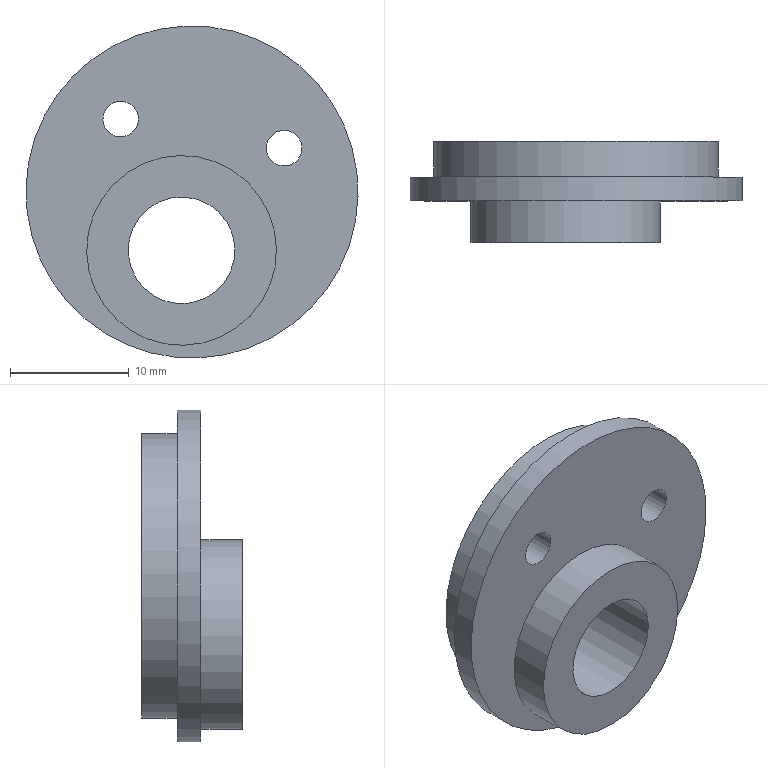Component | NX | ECCENTRIC | 1 solid | 10 faces | box 28 x 8.5 x 28 mm | volume 2681 mm3 | cylinder 6 | plane 4 | commonest cylinder face diameters 3 x2 24 x1 28 x1 16 x1 9 x1
STEP:
#1=CARTESIAN_POINT('',(0.,0.,0.));
#2=DIRECTION('',(0.,0.,1.));
#3=DIRECTION('',(1.,0.,0.));
#4=AXIS2_PLACEMENT_3D('',#1,#2,#3);
#5=CARTESIAN_POINT('',(56.622,60.5,26.855));
#6=VERTEX_POINT('',#5);
#7=CARTESIAN_POINT('',(53.668,60.5,27.381));
#8=VERTEX_POINT('',#7);
#9=CARTESIAN_POINT('',(55.145,60.5,27.118));
#10=DIRECTION('',(0.,-1.,0.));
#11=DIRECTION('',(0.9845,0.,-0.1753));
#12=AXIS2_PLACEMENT_3D('',#9,#10,#11);
#13=CIRCLE('',#12,1.5);
#14=CARTESIAN_POINT('',(47.377,60.5,23.423));
#15=DIRECTION('',(0.,1.,0.));
#16=DIRECTION('',(0.9845,0.,-0.1753));
#17=AXIS2_PLACEMENT_3D('',#14,#15,#16);
#18=PLANE('',#17);
#19=CARTESIAN_POINT('',(8.5,-5.));
#20=CARTESIAN_POINT('',(8.5,-7.598));
#21=CARTESIAN_POINT('',(6.25,-6.299));
#22=CARTESIAN_POINT('',(4.,-5.));
#23=CARTESIAN_POINT('',(6.25,-3.701));
#24=CARTESIAN_POINT('',(8.5,-2.402));
#25=CARTESIAN_POINT('',(8.5,-5.));
#26=(BOUNDED_CURVE()B_SPLINE_CURVE(2,(#19,#20,#21,#22,#23,#24,#25),.UNSPECIFIED.,.T.,.F.)B_SPLINE_CURVE_WITH_KNOTS((1,2,2,2,2,1),(-2.094,0.,2.094,4.189,6.283,8.378),.UNSPECIFIED.)CURVE()GEOMETRIC_REPRESENTATION_ITEM()RATIONAL_B_SPLINE_CURVE((1.,0.5,1.,0.5,1.,0.5,1.))REPRESENTATION_ITEM(''));
#27=(GEOMETRIC_REPRESENTATION_CONTEXT(2)PARAMETRIC_REPRESENTATION_CONTEXT()REPRESENTATION_CONTEXT('',''));
#28=DEFINITIONAL_REPRESENTATION('',(#26),#27);
#29=PCURVE('',#18,#28);
#30=CARTESIAN_POINT('',(55.145,72.,27.118));
#31=DIRECTION('',(0.,-1.,0.));
#32=DIRECTION('',(-0.9845,0.,0.1753));
#33=AXIS2_PLACEMENT_3D('',#30,#31,#32);
#34=CYLINDRICAL_SURFACE('',#33,1.5);
#35=CARTESIAN_POINT('',(3.142,11.5));
#36=DIRECTION('',(1.,0.));
#37=VECTOR('',#36,1.);
#38=LINE('',#35,#37);
#39=(GEOMETRIC_REPRESENTATION_CONTEXT(2)PARAMETRIC_REPRESENTATION_CONTEXT()REPRESENTATION_CONTEXT('',''));
#40=DEFINITIONAL_REPRESENTATION('',(#38),#39);
#41=PCURVE('',#34,#40);
#42=SURFACE_CURVE('',#13,(#29,#41),.PCURVE_S1.);
#43=EDGE_CURVE('',#6,#8,#42,.T.);
#44=ORIENTED_EDGE('',*,*,#43,.T.);
#45=CARTESIAN_POINT('',(55.145,60.5,27.118));
#46=DIRECTION('',(0.,-1.,0.));
#47=DIRECTION('',(0.9845,0.,-0.1753));
#48=AXIS2_PLACEMENT_3D('',#45,#46,#47);
#49=CIRCLE('',#48,1.5);
#50=CARTESIAN_POINT('',(8.5,-5.));
#51=CARTESIAN_POINT('',(8.5,-7.598));
#52=CARTESIAN_POINT('',(6.25,-6.299));
#53=CARTESIAN_POINT('',(4.,-5.));
#54=CARTESIAN_POINT('',(6.25,-3.701));
#55=CARTESIAN_POINT('',(8.5,-2.402));
#56=CARTESIAN_POINT('',(8.5,-5.));
#57=(BOUNDED_CURVE()B_SPLINE_CURVE(2,(#50,#51,#52,#53,#54,#55,#56),.UNSPECIFIED.,.T.,.F.)B_SPLINE_CURVE_WITH_KNOTS((1,2,2,2,2,1),(-2.094,0.,2.094,4.189,6.283,8.378),.UNSPECIFIED.)CURVE()GEOMETRIC_REPRESENTATION_ITEM()RATIONAL_B_SPLINE_CURVE((1.,0.5,1.,0.5,1.,0.5,1.))REPRESENTATION_ITEM(''));
#58=(GEOMETRIC_REPRESENTATION_CONTEXT(2)PARAMETRIC_REPRESENTATION_CONTEXT()REPRESENTATION_CONTEXT('',''));
#59=DEFINITIONAL_REPRESENTATION('',(#57),#58);
#60=PCURVE('',#18,#59);
#61=CARTESIAN_POINT('',(-3.142,11.5));
#62=DIRECTION('',(1.,0.));
#63=VECTOR('',#62,1.);
#64=LINE('',#61,#63);
#65=(GEOMETRIC_REPRESENTATION_CONTEXT(2)PARAMETRIC_REPRESENTATION_CONTEXT()REPRESENTATION_CONTEXT('',''));
#66=DEFINITIONAL_REPRESENTATION('',(#64),#65);
#67=PCURVE('',#34,#66);
#68=SURFACE_CURVE('',#49,(#60,#67),.PCURVE_S1.);
#69=EDGE_CURVE('',#8,#6,#68,.T.);
#70=ORIENTED_EDGE('',*,*,#69,.T.);
#71=EDGE_LOOP('',(#44,#70));
#72=FACE_BOUND('',#71,.T.);
#73=CARTESIAN_POINT('',(50.93,60.5,17.711));
#74=VERTEX_POINT('',#73);
#75=CARTESIAN_POINT('',(42.07,60.5,19.289));
#76=VERTEX_POINT('',#75);
#77=CARTESIAN_POINT('',(46.5,60.5,18.5));
#78=DIRECTION('',(0.,-1.,0.));
#79=DIRECTION('',(0.9845,0.,-0.1753));
#80=AXIS2_PLACEMENT_3D('',#77,#78,#79);
#81=CIRCLE('',#80,4.5);
#82=CARTESIAN_POINT('',(4.5,5.));
#83=CARTESIAN_POINT('',(4.5,-2.794));
#84=CARTESIAN_POINT('',(-2.25,1.103));
#85=CARTESIAN_POINT('',(-9.,5.));
#86=CARTESIAN_POINT('',(-2.25,8.897));
#87=CARTESIAN_POINT('',(4.5,12.794));
#88=CARTESIAN_POINT('',(4.5,5.));
#89=(BOUNDED_CURVE()B_SPLINE_CURVE(2,(#82,#83,#84,#85,#86,#87,#88),.UNSPECIFIED.,.T.,.F.)B_SPLINE_CURVE_WITH_KNOTS((1,2,2,2,2,1),(-2.094,0.,2.094,4.189,6.283,8.378),.UNSPECIFIED.)CURVE()GEOMETRIC_REPRESENTATION_ITEM()RATIONAL_B_SPLINE_CURVE((1.,0.5,1.,0.5,1.,0.5,1.))REPRESENTATION_ITEM(''));
#90=(GEOMETRIC_REPRESENTATION_CONTEXT(2)PARAMETRIC_REPRESENTATION_CONTEXT()REPRESENTATION_CONTEXT('',''));
#91=DEFINITIONAL_REPRESENTATION('',(#89),#90);
#92=PCURVE('',#18,#91);
#93=CARTESIAN_POINT('',(46.5,72.,18.5));
#94=DIRECTION('',(0.,-1.,0.));
#95=DIRECTION('',(-0.9845,0.,0.1753));
#96=AXIS2_PLACEMENT_3D('',#93,#94,#95);
#97=CYLINDRICAL_SURFACE('',#96,4.5);
#98=CARTESIAN_POINT('',(3.142,11.5));
#99=DIRECTION('',(1.,0.));
#100=VECTOR('',#99,1.);
#101=LINE('',#98,#100);
#102=(GEOMETRIC_REPRESENTATION_CONTEXT(2)PARAMETRIC_REPRESENTATION_CONTEXT()REPRESENTATION_CONTEXT('',''));
#103=DEFINITIONAL_REPRESENTATION('',(#101),#102);
#104=PCURVE('',#97,#103);
#105=SURFACE_CURVE('',#81,(#92,#104),.PCURVE_S1.);
#106=EDGE_CURVE('',#74,#76,#105,.T.);
#107=ORIENTED_EDGE('',*,*,#106,.T.);
#108=CARTESIAN_POINT('',(46.5,60.5,18.5));
#109=DIRECTION('',(0.,-1.,0.));
#110=DIRECTION('',(0.9845,0.,-0.1753));
#111=AXIS2_PLACEMENT_3D('',#108,#109,#110);
#112=CIRCLE('',#111,4.5);
#113=CARTESIAN_POINT('',(4.5,5.));
#114=CARTESIAN_POINT('',(4.5,-2.794));
#115=CARTESIAN_POINT('',(-2.25,1.103));
#116=CARTESIAN_POINT('',(-9.,5.));
#117=CARTESIAN_POINT('',(-2.25,8.897));
#118=CARTESIAN_POINT('',(4.5,12.794));
#119=CARTESIAN_POINT('',(4.5,5.));
#120=(BOUNDED_CURVE()B_SPLINE_CURVE(2,(#113,#114,#115,#116,#117,#118,#119),.UNSPECIFIED.,.T.,.F.)B_SPLINE_CURVE_WITH_KNOTS((1,2,2,2,2,1),(-2.094,0.,2.094,4.189,6.283,8.378),.UNSPECIFIED.)CURVE()GEOMETRIC_REPRESENTATION_ITEM()RATIONAL_B_SPLINE_CURVE((1.,0.5,1.,0.5,1.,0.5,1.))REPRESENTATION_ITEM(''));
#121=(GEOMETRIC_REPRESENTATION_CONTEXT(2)PARAMETRIC_REPRESENTATION_CONTEXT()REPRESENTATION_CONTEXT('',''));
#122=DEFINITIONAL_REPRESENTATION('',(#120),#121);
#123=PCURVE('',#18,#122);
#124=CARTESIAN_POINT('',(-3.142,11.5));
#125=DIRECTION('',(1.,0.));
#126=VECTOR('',#125,1.);
#127=LINE('',#124,#126);
#128=(GEOMETRIC_REPRESENTATION_CONTEXT(2)PARAMETRIC_REPRESENTATION_CONTEXT()REPRESENTATION_CONTEXT('',''));
#129=DEFINITIONAL_REPRESENTATION('',(#127),#128);
#130=PCURVE('',#97,#129);
#131=SURFACE_CURVE('',#112,(#123,#130),.PCURVE_S1.);
#132=EDGE_CURVE('',#76,#74,#131,.T.);
#133=ORIENTED_EDGE('',*,*,#132,.T.);
#134=EDGE_LOOP('',(#107,#133));
#135=FACE_BOUND('',#134,.T.);
#136=CARTESIAN_POINT('',(35.563,60.5,25.526));
#137=VERTEX_POINT('',#136);
#138=CARTESIAN_POINT('',(47.377,60.5,23.423));
#139=DIRECTION('',(0.,-1.,0.));
#140=DIRECTION('',(-0.9845,0.,0.1753));
#141=AXIS2_PLACEMENT_3D('',#138,#139,#140);
#142=CIRCLE('',#141,12.);
#143=CARTESIAN_POINT('',(-12.,0.));
#144=CARTESIAN_POINT('',(-12.,20.785));
#145=CARTESIAN_POINT('',(6.,10.392));
#146=CARTESIAN_POINT('',(24.,0.));
#147=CARTESIAN_POINT('',(6.,-10.392));
#148=CARTESIAN_POINT('',(-12.,-20.785));
#149=CARTESIAN_POINT('',(-12.,0.));
#150=(BOUNDED_CURVE()B_SPLINE_CURVE(2,(#143,#144,#145,#146,#147,#148,#149),.UNSPECIFIED.,.T.,.F.)B_SPLINE_CURVE_WITH_KNOTS((1,2,2,2,2,1),(-2.094,0.,2.094,4.189,6.283,8.378),.UNSPECIFIED.)CURVE()GEOMETRIC_REPRESENTATION_ITEM()RATIONAL_B_SPLINE_CURVE((1.,0.5,1.,0.5,1.,0.5,1.))REPRESENTATION_ITEM(''));
#151=(GEOMETRIC_REPRESENTATION_CONTEXT(2)PARAMETRIC_REPRESENTATION_CONTEXT()REPRESENTATION_CONTEXT('',''));
#152=DEFINITIONAL_REPRESENTATION('',(#150),#151);
#153=PCURVE('',#18,#152);
#154=CARTESIAN_POINT('',(47.377,60.5,23.423));
#155=DIRECTION('',(0.,-1.,0.));
#156=DIRECTION('',(-0.9845,0.,0.1753));
#157=AXIS2_PLACEMENT_3D('',#154,#155,#156);
#158=CYLINDRICAL_SURFACE('',#157,12.);
#159=CARTESIAN_POINT('',(0.,0.));
#160=DIRECTION('',(1.,0.));
#161=VECTOR('',#160,1.);
#162=LINE('',#159,#161);
#163=(GEOMETRIC_REPRESENTATION_CONTEXT(2)PARAMETRIC_REPRESENTATION_CONTEXT()REPRESENTATION_CONTEXT('',''));
#164=DEFINITIONAL_REPRESENTATION('',(#162),#163);
#165=PCURVE('',#158,#164);
#166=SURFACE_CURVE('',#142,(#153,#165),.PCURVE_S1.);
#167=EDGE_CURVE('',#137,#137,#166,.T.);
#168=ORIENTED_EDGE('',*,*,#167,.F.);
#169=EDGE_LOOP('',(#168));
#170=FACE_BOUND('',#169,.T.);
#171=CARTESIAN_POINT('',(42.838,60.5,29.309));
#172=VERTEX_POINT('',#171);
#173=CARTESIAN_POINT('',(39.885,60.5,29.835));
#174=VERTEX_POINT('',#173);
#175=CARTESIAN_POINT('',(41.362,60.5,29.572));
#176=DIRECTION('',(0.,1.,0.));
#177=DIRECTION('',(0.9845,0.,-0.1753));
#178=AXIS2_PLACEMENT_3D('',#175,#176,#177);
#179=CIRCLE('',#178,1.5);
#180=CARTESIAN_POINT('',(-7.,-5.));
#181=DIRECTION('',(1.,0.));
#182=AXIS2_PLACEMENT_2D('',#180,#181);
#183=CIRCLE('',#182,1.5);
#184=(GEOMETRIC_REPRESENTATION_CONTEXT(2)PARAMETRIC_REPRESENTATION_CONTEXT()REPRESENTATION_CONTEXT('',''));
#185=DEFINITIONAL_REPRESENTATION('',(#183),#184);
#186=PCURVE('',#18,#185);
#187=CARTESIAN_POINT('',(41.362,72.,29.572));
#188=DIRECTION('',(0.,-1.,0.));
#189=DIRECTION('',(-0.9845,0.,0.1753));
#190=AXIS2_PLACEMENT_3D('',#187,#188,#189);
#191=CYLINDRICAL_SURFACE('',#190,1.5);
#192=CARTESIAN_POINT('',(3.142,11.5));
#193=DIRECTION('',(-1.,0.));
#194=VECTOR('',#193,1.);
#195=LINE('',#192,#194);
#196=(GEOMETRIC_REPRESENTATION_CONTEXT(2)PARAMETRIC_REPRESENTATION_CONTEXT()REPRESENTATION_CONTEXT('',''));
#197=DEFINITIONAL_REPRESENTATION('',(#195),#196);
#198=PCURVE('',#191,#197);
#199=SURFACE_CURVE('',#179,(#186,#198),.PCURVE_S1.);
#200=EDGE_CURVE('',#172,#174,#199,.T.);
#201=ORIENTED_EDGE('',*,*,#200,.F.);
#202=CARTESIAN_POINT('',(41.362,60.5,29.572));
#203=DIRECTION('',(0.,1.,0.));
#204=DIRECTION('',(0.9845,0.,-0.1753));
#205=AXIS2_PLACEMENT_3D('',#202,#203,#204);
#206=CIRCLE('',#205,1.5);
#207=CARTESIAN_POINT('',(-7.,-5.));
#208=DIRECTION('',(1.,0.));
#209=AXIS2_PLACEMENT_2D('',#207,#208);
#210=CIRCLE('',#209,1.5);
#211=(GEOMETRIC_REPRESENTATION_CONTEXT(2)PARAMETRIC_REPRESENTATION_CONTEXT()REPRESENTATION_CONTEXT('',''));
#212=DEFINITIONAL_REPRESENTATION('',(#210),#211);
#213=PCURVE('',#18,#212);
#214=CARTESIAN_POINT('',(9.425,11.5));
#215=DIRECTION('',(-1.,0.));
#216=VECTOR('',#215,1.);
#217=LINE('',#214,#216);
#218=(GEOMETRIC_REPRESENTATION_CONTEXT(2)PARAMETRIC_REPRESENTATION_CONTEXT()REPRESENTATION_CONTEXT('',''));
#219=DEFINITIONAL_REPRESENTATION('',(#217),#218);
#220=PCURVE('',#191,#219);
#221=SURFACE_CURVE('',#206,(#213,#220),.PCURVE_S1.);
#222=EDGE_CURVE('',#174,#172,#221,.T.);
#223=ORIENTED_EDGE('',*,*,#222,.F.);
#224=EDGE_LOOP('',(#201,#223));
#225=FACE_BOUND('',#224,.T.);
#226=ADVANCED_FACE('',(#72,#135,#170,#225),#18,.T.);
#227=CARTESIAN_POINT('',(53.668,55.5,27.381));
#228=VERTEX_POINT('',#227);
#229=CARTESIAN_POINT('',(55.145,55.5,27.118));
#230=DIRECTION('',(0.,1.,0.));
#231=DIRECTION('',(-0.9845,0.,0.1753));
#232=AXIS2_PLACEMENT_3D('',#229,#230,#231);
#233=CIRCLE('',#232,1.5);
#234=CARTESIAN_POINT('',(47.377,55.5,23.423));
#235=DIRECTION('',(0.,-1.,0.));
#236=DIRECTION('',(-0.9845,0.,0.1753));
#237=AXIS2_PLACEMENT_3D('',#234,#235,#236);
#238=PLANE('',#237);
#239=CARTESIAN_POINT('',(-5.5,-5.));
#240=CARTESIAN_POINT('',(-5.5,-7.598));
#241=CARTESIAN_POINT('',(-7.75,-6.299));
#242=CARTESIAN_POINT('',(-10.,-5.));
#243=CARTESIAN_POINT('',(-7.75,-3.701));
#244=CARTESIAN_POINT('',(-5.5,-2.402));
#245=CARTESIAN_POINT('',(-5.5,-5.));
#246=(BOUNDED_CURVE()B_SPLINE_CURVE(2,(#239,#240,#241,#242,#243,#244,#245),.UNSPECIFIED.,.T.,.F.)B_SPLINE_CURVE_WITH_KNOTS((1,2,2,2,2,1),(-2.094,0.,2.094,4.189,6.283,8.378),.UNSPECIFIED.)CURVE()GEOMETRIC_REPRESENTATION_ITEM()RATIONAL_B_SPLINE_CURVE((1.,0.5,1.,0.5,1.,0.5,1.))REPRESENTATION_ITEM(''));
#247=(GEOMETRIC_REPRESENTATION_CONTEXT(2)PARAMETRIC_REPRESENTATION_CONTEXT()REPRESENTATION_CONTEXT('',''));
#248=DEFINITIONAL_REPRESENTATION('',(#246),#247);
#249=PCURVE('',#238,#248);
#250=CARTESIAN_POINT('',(6.283,16.5));
#251=DIRECTION('',(-1.,0.));
#252=VECTOR('',#251,1.);
#253=LINE('',#250,#252);
#254=(GEOMETRIC_REPRESENTATION_CONTEXT(2)PARAMETRIC_REPRESENTATION_CONTEXT()REPRESENTATION_CONTEXT('',''));
#255=DEFINITIONAL_REPRESENTATION('',(#253),#254);
#256=PCURVE('',#34,#255);
#257=SURFACE_CURVE('',#233,(#249,#256),.PCURVE_S1.);
#258=EDGE_CURVE('',#228,#228,#257,.T.);
#259=ORIENTED_EDGE('',*,*,#258,.T.);
#260=EDGE_LOOP('',(#259));
#261=FACE_BOUND('',#260,.T.);
#262=CARTESIAN_POINT('',(38.624,55.5,19.903));
#263=VERTEX_POINT('',#262);
#264=CARTESIAN_POINT('',(46.5,55.5,18.5));
#265=DIRECTION('',(0.,-1.,0.));
#266=DIRECTION('',(-0.9845,0.,0.1753));
#267=AXIS2_PLACEMENT_3D('',#264,#265,#266);
#268=CIRCLE('',#267,8.);
#269=CARTESIAN_POINT('',(-0.,5.));
#270=DIRECTION('',(1.,0.));
#271=AXIS2_PLACEMENT_2D('',#269,#270);
#272=CIRCLE('',#271,8.);
#273=(GEOMETRIC_REPRESENTATION_CONTEXT(2)PARAMETRIC_REPRESENTATION_CONTEXT()REPRESENTATION_CONTEXT('',''));
#274=DEFINITIONAL_REPRESENTATION('',(#272),#273);
#275=PCURVE('',#238,#274);
#276=CARTESIAN_POINT('',(46.5,52.,18.5));
#277=DIRECTION('',(0.,1.,0.));
#278=DIRECTION('',(0.9845,0.,-0.1753));
#279=AXIS2_PLACEMENT_3D('',#276,#277,#278);
#280=CYLINDRICAL_SURFACE('',#279,8.);
#281=CARTESIAN_POINT('',(9.425,3.5));
#282=DIRECTION('',(-1.,0.));
#283=VECTOR('',#282,1.);
#284=LINE('',#281,#283);
#285=(GEOMETRIC_REPRESENTATION_CONTEXT(2)PARAMETRIC_REPRESENTATION_CONTEXT()REPRESENTATION_CONTEXT('',''));
#286=DEFINITIONAL_REPRESENTATION('',(#284),#285);
#287=PCURVE('',#280,#286);
#288=SURFACE_CURVE('',#268,(#275,#287),.PCURVE_S1.);
#289=EDGE_CURVE('',#263,#263,#288,.T.);
#290=ORIENTED_EDGE('',*,*,#289,.F.);
#291=EDGE_LOOP('',(#290));
#292=FACE_BOUND('',#291,.T.);
#293=CARTESIAN_POINT('',(33.593,55.5,25.877));
#294=VERTEX_POINT('',#293);
#295=CARTESIAN_POINT('',(47.377,55.5,23.423));
#296=DIRECTION('',(0.,-1.,0.));
#297=DIRECTION('',(-0.9845,0.,0.1753));
#298=AXIS2_PLACEMENT_3D('',#295,#296,#297);
#299=CIRCLE('',#298,14.);
#300=CARTESIAN_POINT('',(0.,0.));
#301=DIRECTION('',(1.,-0.));
#302=AXIS2_PLACEMENT_2D('',#300,#301);
#303=CIRCLE('',#302,14.);
#304=(GEOMETRIC_REPRESENTATION_CONTEXT(2)PARAMETRIC_REPRESENTATION_CONTEXT()REPRESENTATION_CONTEXT('',''));
#305=DEFINITIONAL_REPRESENTATION('',(#303),#304);
#306=PCURVE('',#238,#305);
#307=CARTESIAN_POINT('',(47.377,57.5,23.423));
#308=DIRECTION('',(0.,-1.,0.));
#309=DIRECTION('',(-0.9845,0.,0.1753));
#310=AXIS2_PLACEMENT_3D('',#307,#308,#309);
#311=CYLINDRICAL_SURFACE('',#310,14.);
#312=CARTESIAN_POINT('',(0.,2.));
#313=DIRECTION('',(1.,0.));
#314=VECTOR('',#313,1.);
#315=LINE('',#312,#314);
#316=(GEOMETRIC_REPRESENTATION_CONTEXT(2)PARAMETRIC_REPRESENTATION_CONTEXT()REPRESENTATION_CONTEXT('',''));
#317=DEFINITIONAL_REPRESENTATION('',(#315),#316);
#318=PCURVE('',#311,#317);
#319=SURFACE_CURVE('',#299,(#306,#318),.PCURVE_S1.);
#320=EDGE_CURVE('',#294,#294,#319,.T.);
#321=ORIENTED_EDGE('',*,*,#320,.T.);
#322=EDGE_LOOP('',(#321));
#323=FACE_BOUND('',#322,.T.);
#324=CARTESIAN_POINT('',(39.885,55.5,29.835));
#325=VERTEX_POINT('',#324);
#326=CARTESIAN_POINT('',(41.362,55.5,29.572));
#327=DIRECTION('',(0.,-1.,0.));
#328=DIRECTION('',(-0.9845,0.,0.1753));
#329=AXIS2_PLACEMENT_3D('',#326,#327,#328);
#330=CIRCLE('',#329,1.5);
#331=CARTESIAN_POINT('',(7.,-5.));
#332=DIRECTION('',(1.,-0.));
#333=AXIS2_PLACEMENT_2D('',#331,#332);
#334=CIRCLE('',#333,1.5);
#335=(GEOMETRIC_REPRESENTATION_CONTEXT(2)PARAMETRIC_REPRESENTATION_CONTEXT()REPRESENTATION_CONTEXT('',''));
#336=DEFINITIONAL_REPRESENTATION('',(#334),#335);
#337=PCURVE('',#238,#336);
#338=CARTESIAN_POINT('',(0.,16.5));
#339=DIRECTION('',(1.,0.));
#340=VECTOR('',#339,1.);
#341=LINE('',#338,#340);
#342=(GEOMETRIC_REPRESENTATION_CONTEXT(2)PARAMETRIC_REPRESENTATION_CONTEXT()REPRESENTATION_CONTEXT('',''));
#343=DEFINITIONAL_REPRESENTATION('',(#341),#342);
#344=PCURVE('',#191,#343);
#345=SURFACE_CURVE('',#330,(#337,#344),.PCURVE_S1.);
#346=EDGE_CURVE('',#325,#325,#345,.T.);
#347=ORIENTED_EDGE('',*,*,#346,.F.);
#348=EDGE_LOOP('',(#347));
#349=FACE_BOUND('',#348,.T.);
#350=ADVANCED_FACE('',(#261,#292,#323,#349),#238,.T.);
#351=CARTESIAN_POINT('',(35.563,57.5,25.526));
#352=VERTEX_POINT('',#351);
#353=CARTESIAN_POINT('',(47.377,57.5,23.423));
#354=DIRECTION('',(0.,1.,0.));
#355=DIRECTION('',(-0.9845,0.,0.1753));
#356=AXIS2_PLACEMENT_3D('',#353,#354,#355);
#357=CIRCLE('',#356,12.);
#358=CARTESIAN_POINT('',(6.283,3.));
#359=DIRECTION('',(-1.,0.));
#360=VECTOR('',#359,1.);
#361=LINE('',#358,#360);
#362=(GEOMETRIC_REPRESENTATION_CONTEXT(2)PARAMETRIC_REPRESENTATION_CONTEXT()REPRESENTATION_CONTEXT('',''));
#363=DEFINITIONAL_REPRESENTATION('',(#361),#362);
#364=PCURVE('',#158,#363);
#365=CARTESIAN_POINT('',(47.377,57.5,23.423));
#366=DIRECTION('',(0.,1.,0.));
#367=DIRECTION('',(0.9845,0.,-0.1753));
#368=AXIS2_PLACEMENT_3D('',#365,#366,#367);
#369=PLANE('',#368);
#370=CARTESIAN_POINT('',(0.,0.));
#371=DIRECTION('',(-1.,0.));
#372=AXIS2_PLACEMENT_2D('',#370,#371);
#373=CIRCLE('',#372,12.);
#374=(GEOMETRIC_REPRESENTATION_CONTEXT(2)PARAMETRIC_REPRESENTATION_CONTEXT()REPRESENTATION_CONTEXT('',''));
#375=DEFINITIONAL_REPRESENTATION('',(#373),#374);
#376=PCURVE('',#369,#375);
#377=SURFACE_CURVE('',#357,(#364,#376),.PCURVE_S1.);
#378=EDGE_CURVE('',#352,#352,#377,.T.);
#379=ORIENTED_EDGE('',*,*,#378,.T.);
#380=CARTESIAN_POINT('',(35.563,60.5,25.526));
#381=CARTESIAN_POINT('',(35.563,57.5,25.526));
#382=B_SPLINE_CURVE_WITH_KNOTS('',1,(#380,#381),.UNSPECIFIED.,.F.,.F.,(2,2),(0.,3.),.PIECEWISE_BEZIER_KNOTS.);
#383=CARTESIAN_POINT('',(0.,0.));
#384=DIRECTION('',(0.,1.));
#385=VECTOR('',#384,1.);
#386=LINE('',#383,#385);
#387=(GEOMETRIC_REPRESENTATION_CONTEXT(2)PARAMETRIC_REPRESENTATION_CONTEXT()REPRESENTATION_CONTEXT('',''));
#388=DEFINITIONAL_REPRESENTATION('',(#386),#387);
#389=PCURVE('',#158,#388);
#390=CARTESIAN_POINT('',(6.283,0.));
#391=DIRECTION('',(0.,1.));
#392=VECTOR('',#391,1.);
#393=LINE('',#390,#392);
#394=(GEOMETRIC_REPRESENTATION_CONTEXT(2)PARAMETRIC_REPRESENTATION_CONTEXT()REPRESENTATION_CONTEXT('',''));
#395=DEFINITIONAL_REPRESENTATION('',(#393),#394);
#396=PCURVE('',#158,#395);
#397=SEAM_CURVE('',#382,(#389,#396),.PCURVE_S1.);
#398=EDGE_CURVE('',#137,#352,#397,.T.);
#399=ORIENTED_EDGE('',*,*,#398,.F.);
#400=ORIENTED_EDGE('',*,*,#167,.T.);
#401=ORIENTED_EDGE('',*,*,#398,.T.);
#402=EDGE_LOOP('',(#379,#399,#400,#401));
#403=FACE_BOUND('',#402,.T.);
#404=ADVANCED_FACE('',(#403),#158,.T.);
#405=ORIENTED_EDGE('',*,*,#378,.F.);
#406=EDGE_LOOP('',(#405));
#407=FACE_BOUND('',#406,.T.);
#408=CARTESIAN_POINT('',(33.593,57.5,25.877));
#409=VERTEX_POINT('',#408);
#410=CARTESIAN_POINT('',(47.377,57.5,23.423));
#411=DIRECTION('',(0.,-1.,0.));
#412=DIRECTION('',(-0.9845,0.,0.1753));
#413=AXIS2_PLACEMENT_3D('',#410,#411,#412);
#414=CIRCLE('',#413,14.);
#415=CARTESIAN_POINT('',(-14.,-0.));
#416=CARTESIAN_POINT('',(-14.,24.249));
#417=CARTESIAN_POINT('',(7.,12.124));
#418=CARTESIAN_POINT('',(28.,0.));
#419=CARTESIAN_POINT('',(7.,-12.124));
#420=CARTESIAN_POINT('',(-14.,-24.249));
#421=CARTESIAN_POINT('',(-14.,-0.));
#422=(BOUNDED_CURVE()B_SPLINE_CURVE(2,(#415,#416,#417,#418,#419,#420,#421),.UNSPECIFIED.,.T.,.F.)B_SPLINE_CURVE_WITH_KNOTS((1,2,2,2,2,1),(-2.094,0.,2.094,4.189,6.283,8.378),.UNSPECIFIED.)CURVE()GEOMETRIC_REPRESENTATION_ITEM()RATIONAL_B_SPLINE_CURVE((1.,0.5,1.,0.5,1.,0.5,1.))REPRESENTATION_ITEM(''));
#423=(GEOMETRIC_REPRESENTATION_CONTEXT(2)PARAMETRIC_REPRESENTATION_CONTEXT()REPRESENTATION_CONTEXT('',''));
#424=DEFINITIONAL_REPRESENTATION('',(#422),#423);
#425=PCURVE('',#369,#424);
#426=CARTESIAN_POINT('',(0.,0.));
#427=DIRECTION('',(1.,0.));
#428=VECTOR('',#427,1.);
#429=LINE('',#426,#428);
#430=(GEOMETRIC_REPRESENTATION_CONTEXT(2)PARAMETRIC_REPRESENTATION_CONTEXT()REPRESENTATION_CONTEXT('',''));
#431=DEFINITIONAL_REPRESENTATION('',(#429),#430);
#432=PCURVE('',#311,#431);
#433=SURFACE_CURVE('',#414,(#425,#432),.PCURVE_S1.);
#434=EDGE_CURVE('',#409,#409,#433,.T.);
#435=ORIENTED_EDGE('',*,*,#434,.F.);
#436=EDGE_LOOP('',(#435));
#437=FACE_BOUND('',#436,.T.);
#438=ADVANCED_FACE('',(#407,#437),#369,.T.);
#439=ORIENTED_EDGE('',*,*,#320,.F.);
#440=CARTESIAN_POINT('',(33.593,57.5,25.877));
#441=CARTESIAN_POINT('',(33.593,55.5,25.877));
#442=B_SPLINE_CURVE_WITH_KNOTS('',1,(#440,#441),.UNSPECIFIED.,.F.,.F.,(2,2),(0.,2.),.PIECEWISE_BEZIER_KNOTS.);
#443=CARTESIAN_POINT('',(0.,0.));
#444=DIRECTION('',(0.,1.));
#445=VECTOR('',#444,1.);
#446=LINE('',#443,#445);
#447=(GEOMETRIC_REPRESENTATION_CONTEXT(2)PARAMETRIC_REPRESENTATION_CONTEXT()REPRESENTATION_CONTEXT('',''));
#448=DEFINITIONAL_REPRESENTATION('',(#446),#447);
#449=PCURVE('',#311,#448);
#450=CARTESIAN_POINT('',(6.283,0.));
#451=DIRECTION('',(0.,1.));
#452=VECTOR('',#451,1.);
#453=LINE('',#450,#452);
#454=(GEOMETRIC_REPRESENTATION_CONTEXT(2)PARAMETRIC_REPRESENTATION_CONTEXT()REPRESENTATION_CONTEXT('',''));
#455=DEFINITIONAL_REPRESENTATION('',(#453),#454);
#456=PCURVE('',#311,#455);
#457=SEAM_CURVE('',#442,(#449,#456),.PCURVE_S1.);
#458=EDGE_CURVE('',#409,#294,#457,.T.);
#459=ORIENTED_EDGE('',*,*,#458,.F.);
#460=ORIENTED_EDGE('',*,*,#434,.T.);
#461=ORIENTED_EDGE('',*,*,#458,.T.);
#462=EDGE_LOOP('',(#439,#459,#460,#461));
#463=FACE_BOUND('',#462,.T.);
#464=ADVANCED_FACE('',(#463),#311,.T.);
#465=CARTESIAN_POINT('',(38.624,52.,19.903));
#466=VERTEX_POINT('',#465);
#467=CARTESIAN_POINT('',(46.5,52.,18.5));
#468=DIRECTION('',(0.,-1.,0.));
#469=DIRECTION('',(-0.9845,0.,0.1753));
#470=AXIS2_PLACEMENT_3D('',#467,#468,#469);
#471=CIRCLE('',#470,8.);
#472=CARTESIAN_POINT('',(9.425,0.));
#473=DIRECTION('',(-1.,0.));
#474=VECTOR('',#473,1.);
#475=LINE('',#472,#474);
#476=(GEOMETRIC_REPRESENTATION_CONTEXT(2)PARAMETRIC_REPRESENTATION_CONTEXT()REPRESENTATION_CONTEXT('',''));
#477=DEFINITIONAL_REPRESENTATION('',(#475),#476);
#478=PCURVE('',#280,#477);
#479=CARTESIAN_POINT('',(46.5,52.,18.5));
#480=DIRECTION('',(0.,-1.,0.));
#481=DIRECTION('',(-0.9845,0.,0.1753));
#482=AXIS2_PLACEMENT_3D('',#479,#480,#481);
#483=PLANE('',#482);
#484=CARTESIAN_POINT('',(0.,0.));
#485=DIRECTION('',(1.,0.));
#486=AXIS2_PLACEMENT_2D('',#484,#485);
#487=CIRCLE('',#486,8.);
#488=(GEOMETRIC_REPRESENTATION_CONTEXT(2)PARAMETRIC_REPRESENTATION_CONTEXT()REPRESENTATION_CONTEXT('',''));
#489=DEFINITIONAL_REPRESENTATION('',(#487),#488);
#490=PCURVE('',#483,#489);
#491=SURFACE_CURVE('',#471,(#478,#490),.PCURVE_S1.);
#492=EDGE_CURVE('',#466,#466,#491,.T.);
#493=ORIENTED_EDGE('',*,*,#492,.F.);
#494=CARTESIAN_POINT('',(38.624,52.,19.903));
#495=CARTESIAN_POINT('',(38.624,55.5,19.903));
#496=B_SPLINE_CURVE_WITH_KNOTS('',1,(#494,#495),.UNSPECIFIED.,.F.,.F.,(2,2),(0.,3.5),.PIECEWISE_BEZIER_KNOTS.);
#497=CARTESIAN_POINT('',(9.425,0.));
#498=DIRECTION('',(0.,1.));
#499=VECTOR('',#498,1.);
#500=LINE('',#497,#499);
#501=(GEOMETRIC_REPRESENTATION_CONTEXT(2)PARAMETRIC_REPRESENTATION_CONTEXT()REPRESENTATION_CONTEXT('',''));
#502=DEFINITIONAL_REPRESENTATION('',(#500),#501);
#503=PCURVE('',#280,#502);
#504=CARTESIAN_POINT('',(3.142,0.));
#505=DIRECTION('',(0.,1.));
#506=VECTOR('',#505,1.);
#507=LINE('',#504,#506);
#508=(GEOMETRIC_REPRESENTATION_CONTEXT(2)PARAMETRIC_REPRESENTATION_CONTEXT()REPRESENTATION_CONTEXT('',''));
#509=DEFINITIONAL_REPRESENTATION('',(#507),#508);
#510=PCURVE('',#280,#509);
#511=SEAM_CURVE('',#496,(#503,#510),.PCURVE_S1.);
#512=EDGE_CURVE('',#466,#263,#511,.T.);
#513=ORIENTED_EDGE('',*,*,#512,.T.);
#514=ORIENTED_EDGE('',*,*,#289,.T.);
#515=ORIENTED_EDGE('',*,*,#512,.F.);
#516=EDGE_LOOP('',(#493,#513,#514,#515));
#517=FACE_BOUND('',#516,.T.);
#518=ADVANCED_FACE('',(#517),#280,.T.);
#519=CARTESIAN_POINT('',(42.07,52.,19.289));
#520=VERTEX_POINT('',#519);
#521=CARTESIAN_POINT('',(46.5,52.,18.5));
#522=DIRECTION('',(0.,1.,0.));
#523=DIRECTION('',(-0.9845,0.,0.1753));
#524=AXIS2_PLACEMENT_3D('',#521,#522,#523);
#525=CIRCLE('',#524,4.5);
#526=CARTESIAN_POINT('',(4.5,0.));
#527=CARTESIAN_POINT('',(4.5,-7.794));
#528=CARTESIAN_POINT('',(-2.25,-3.897));
#529=CARTESIAN_POINT('',(-9.,-0.));
#530=CARTESIAN_POINT('',(-2.25,3.897));
#531=CARTESIAN_POINT('',(4.5,7.794));
#532=CARTESIAN_POINT('',(4.5,0.));
#533=(BOUNDED_CURVE()B_SPLINE_CURVE(2,(#526,#527,#528,#529,#530,#531,#532),.UNSPECIFIED.,.T.,.F.)B_SPLINE_CURVE_WITH_KNOTS((1,2,2,2,2,1),(-2.094,0.,2.094,4.189,6.283,8.378),.UNSPECIFIED.)CURVE()GEOMETRIC_REPRESENTATION_ITEM()RATIONAL_B_SPLINE_CURVE((1.,0.5,1.,0.5,1.,0.5,1.))REPRESENTATION_ITEM(''));
#534=(GEOMETRIC_REPRESENTATION_CONTEXT(2)PARAMETRIC_REPRESENTATION_CONTEXT()REPRESENTATION_CONTEXT('',''));
#535=DEFINITIONAL_REPRESENTATION('',(#533),#534);
#536=PCURVE('',#483,#535);
#537=CARTESIAN_POINT('',(6.283,20.));
#538=DIRECTION('',(-1.,0.));
#539=VECTOR('',#538,1.);
#540=LINE('',#537,#539);
#541=(GEOMETRIC_REPRESENTATION_CONTEXT(2)PARAMETRIC_REPRESENTATION_CONTEXT()REPRESENTATION_CONTEXT('',''));
#542=DEFINITIONAL_REPRESENTATION('',(#540),#541);
#543=PCURVE('',#97,#542);
#544=SURFACE_CURVE('',#525,(#536,#543),.PCURVE_S1.);
#545=EDGE_CURVE('',#520,#520,#544,.T.);
#546=ORIENTED_EDGE('',*,*,#545,.T.);
#547=EDGE_LOOP('',(#546));
#548=FACE_BOUND('',#547,.T.);
#549=ORIENTED_EDGE('',*,*,#492,.T.);
#550=EDGE_LOOP('',(#549));
#551=FACE_BOUND('',#550,.T.);
#552=ADVANCED_FACE('',(#548,#551),#483,.T.);
#553=ORIENTED_EDGE('',*,*,#43,.T.);
#554=CARTESIAN_POINT('',(53.668,60.5,27.381));
#555=CARTESIAN_POINT('',(53.668,55.5,27.381));
#556=B_SPLINE_CURVE_WITH_KNOTS('',1,(#554,#555),.UNSPECIFIED.,.F.,.F.,(2,2),(11.5,16.5),.PIECEWISE_BEZIER_KNOTS.);
#557=CARTESIAN_POINT('',(6.283,0.));
#558=DIRECTION('',(0.,1.));
#559=VECTOR('',#558,1.);
#560=LINE('',#557,#559);
#561=(GEOMETRIC_REPRESENTATION_CONTEXT(2)PARAMETRIC_REPRESENTATION_CONTEXT()REPRESENTATION_CONTEXT('',''));
#562=DEFINITIONAL_REPRESENTATION('',(#560),#561);
#563=PCURVE('',#34,#562);
#564=CARTESIAN_POINT('',(0.,0.));
#565=DIRECTION('',(0.,1.));
#566=VECTOR('',#565,1.);
#567=LINE('',#564,#566);
#568=(GEOMETRIC_REPRESENTATION_CONTEXT(2)PARAMETRIC_REPRESENTATION_CONTEXT()REPRESENTATION_CONTEXT('',''));
#569=DEFINITIONAL_REPRESENTATION('',(#567),#568);
#570=PCURVE('',#34,#569);
#571=SEAM_CURVE('',#556,(#563,#570),.PCURVE_S1.);
#572=EDGE_CURVE('',#8,#228,#571,.T.);
#573=ORIENTED_EDGE('',*,*,#572,.T.);
#574=ORIENTED_EDGE('',*,*,#258,.T.);
#575=ORIENTED_EDGE('',*,*,#572,.F.);
#576=ORIENTED_EDGE('',*,*,#69,.T.);
#577=EDGE_LOOP('',(#553,#573,#574,#575,#576));
#578=FACE_BOUND('',#577,.F.);
#579=ADVANCED_FACE('',(#578),#34,.F.);
#580=ORIENTED_EDGE('',*,*,#222,.F.);
#581=CARTESIAN_POINT('',(39.885,60.5,29.835));
#582=CARTESIAN_POINT('',(39.885,55.5,29.835));
#583=B_SPLINE_CURVE_WITH_KNOTS('',1,(#581,#582),.UNSPECIFIED.,.F.,.F.,(2,2),(11.5,16.5),.PIECEWISE_BEZIER_KNOTS.);
#584=CARTESIAN_POINT('',(6.283,0.));
#585=DIRECTION('',(0.,1.));
#586=VECTOR('',#585,1.);
#587=LINE('',#584,#586);
#588=(GEOMETRIC_REPRESENTATION_CONTEXT(2)PARAMETRIC_REPRESENTATION_CONTEXT()REPRESENTATION_CONTEXT('',''));
#589=DEFINITIONAL_REPRESENTATION('',(#587),#588);
#590=PCURVE('',#191,#589);
#591=CARTESIAN_POINT('',(0.,0.));
#592=DIRECTION('',(0.,1.));
#593=VECTOR('',#592,1.);
#594=LINE('',#591,#593);
#595=(GEOMETRIC_REPRESENTATION_CONTEXT(2)PARAMETRIC_REPRESENTATION_CONTEXT()REPRESENTATION_CONTEXT('',''));
#596=DEFINITIONAL_REPRESENTATION('',(#594),#595);
#597=PCURVE('',#191,#596);
#598=SEAM_CURVE('',#583,(#590,#597),.PCURVE_S1.);
#599=EDGE_CURVE('',#174,#325,#598,.T.);
#600=ORIENTED_EDGE('',*,*,#599,.T.);
#601=ORIENTED_EDGE('',*,*,#346,.F.);
#602=ORIENTED_EDGE('',*,*,#599,.F.);
#603=ORIENTED_EDGE('',*,*,#200,.F.);
#604=EDGE_LOOP('',(#580,#600,#601,#602,#603));
#605=FACE_BOUND('',#604,.F.);
#606=ADVANCED_FACE('',(#605),#191,.F.);
#607=ORIENTED_EDGE('',*,*,#106,.T.);
#608=CARTESIAN_POINT('',(42.07,60.5,19.289));
#609=CARTESIAN_POINT('',(42.07,52.,19.289));
#610=B_SPLINE_CURVE_WITH_KNOTS('',1,(#608,#609),.UNSPECIFIED.,.F.,.F.,(2,2),(11.5,20.),.PIECEWISE_BEZIER_KNOTS.);
#611=CARTESIAN_POINT('',(6.283,0.));
#612=DIRECTION('',(0.,1.));
#613=VECTOR('',#612,1.);
#614=LINE('',#611,#613);
#615=(GEOMETRIC_REPRESENTATION_CONTEXT(2)PARAMETRIC_REPRESENTATION_CONTEXT()REPRESENTATION_CONTEXT('',''));
#616=DEFINITIONAL_REPRESENTATION('',(#614),#615);
#617=PCURVE('',#97,#616);
#618=CARTESIAN_POINT('',(0.,0.));
#619=DIRECTION('',(0.,1.));
#620=VECTOR('',#619,1.);
#621=LINE('',#618,#620);
#622=(GEOMETRIC_REPRESENTATION_CONTEXT(2)PARAMETRIC_REPRESENTATION_CONTEXT()REPRESENTATION_CONTEXT('',''));
#623=DEFINITIONAL_REPRESENTATION('',(#621),#622);
#624=PCURVE('',#97,#623);
#625=SEAM_CURVE('',#610,(#617,#624),.PCURVE_S1.);
#626=EDGE_CURVE('',#76,#520,#625,.T.);
#627=ORIENTED_EDGE('',*,*,#626,.T.);
#628=ORIENTED_EDGE('',*,*,#545,.T.);
#629=ORIENTED_EDGE('',*,*,#626,.F.);
#630=ORIENTED_EDGE('',*,*,#132,.T.);
#631=EDGE_LOOP('',(#607,#627,#628,#629,#630));
#632=FACE_BOUND('',#631,.F.);
#633=ADVANCED_FACE('',(#632),#97,.F.);
#634=CLOSED_SHELL('',(#226,#350,#404,#438,#464,#518,#552,#579,#606,#633));
#635=MANIFOLD_SOLID_BREP('',#634);
#636=(LENGTH_UNIT()NAMED_UNIT(*)SI_UNIT(.MILLI.,.METRE.));
#637=UNCERTAINTY_MEASURE_WITH_UNIT(LENGTH_MEASURE(0.000005),#636,'','');
#638=(NAMED_UNIT(*)PLANE_ANGLE_UNIT()SI_UNIT($,.RADIAN.));
#639=(NAMED_UNIT(*)SI_UNIT($,.STERADIAN.)SOLID_ANGLE_UNIT());
#640=(GEOMETRIC_REPRESENTATION_CONTEXT(3)GLOBAL_UNCERTAINTY_ASSIGNED_CONTEXT((#637))GLOBAL_UNIT_ASSIGNED_CONTEXT((#636,#638,#639))REPRESENTATION_CONTEXT('',''));
#641=ADVANCED_BREP_SHAPE_REPRESENTATION('',(#4,#635),#640);